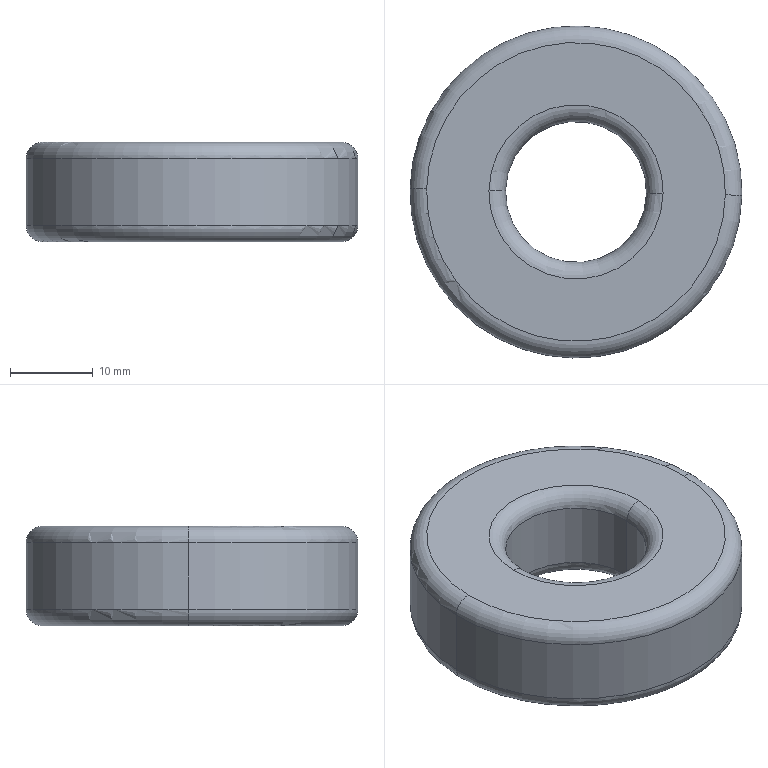Component | SolidWorks | NewCurveBender6203Bearing-DoubleWheel-1 | 1 solid | 14 faces | box 40 x 40 x 12 mm | volume 12048 mm3 | torus 8 | cylinder 4 | plane 2 | commonest cylinder face diameters 17 x2 40 x2
build123d program:
from build123d import *

# Parameters (mm, degrees)
SKETCH1_R           = 20
SKETCH1_R_2         = 8.5
BOSS_EXTRUDE1_DEPTH = 12
FILLET1_R           = 2


with BuildPart() as part:
    # Sketch1 → Boss-Extrude1 (new body)
    with BuildSketch(Plane.XY):
        Circle(SKETCH1_R)
        Circle(SKETCH1_R_2, mode=Mode.SUBTRACT)
    extrude(amount=BOSS_EXTRUDE1_DEPTH)

    # Fillet1
    fillet1_edges = [part.edges().sort_by_distance(p)[0] for p in [
        (-20, 0, 0),
        (-20, 0, 12),
        (-8.5, 0, 0),
        (-8.5, 0, 12),
    ]]
    fillet(fillet1_edges, radius=FILLET1_R)


solid = part.part

# Placed as in the assembly
solid = solid.moved(Location((0, -50.5, 47), (0, 0, 0)))
STEP:
#1=COLOUR_RGB('',0.7922,0.8196,0.9333);
#2=FILL_AREA_STYLE_COLOUR('',#1);
#3=FILL_AREA_STYLE('',(#2));
#4=SURFACE_STYLE_FILL_AREA(#3);
#5=SURFACE_SIDE_STYLE('',(#4));
#6=SURFACE_STYLE_USAGE(.BOTH.,#5);
#7=PRESENTATION_STYLE_ASSIGNMENT((#6));
#8=CARTESIAN_POINT('',(-0.7872,-1.973,2.244));
#9=VERTEX_POINT('',#8);
#10=CARTESIAN_POINT('',(0.7872,-2.004,2.244));
#11=VERTEX_POINT('',#10);
#12=CARTESIAN_POINT('',(0.,-1.988,2.244));
#13=DIRECTION('',(0.,0.,-1.));
#14=DIRECTION('',(0.9998,-0.01988,0.));
#15=AXIS2_PLACEMENT_3D('',#12,#13,#14);
#16=CIRCLE('',#15,0.7874);
#17=EDGE_CURVE('',#9,#11,#16,.T.);
#18=ORIENTED_EDGE('',*,*,#17,.F.);
#19=CARTESIAN_POINT('',(-0.7085,-1.974,2.323));
#20=VERTEX_POINT('',#19);
#21=CARTESIAN_POINT('',(-0.7085,-1.974,2.244));
#22=DIRECTION('',(0.01988,0.9998,0.));
#23=DIRECTION('',(-0.9998,0.01988,0.));
#24=AXIS2_PLACEMENT_3D('',#21,#22,#23);
#25=CIRCLE('',#24,0.07874);
#26=EDGE_CURVE('',#9,#20,#25,.T.);
#27=ORIENTED_EDGE('',*,*,#26,.T.);
#28=CARTESIAN_POINT('',(0.7085,-2.002,2.323));
#29=VERTEX_POINT('',#28);
#30=CARTESIAN_POINT('',(0.,-1.988,2.323));
#31=DIRECTION('',(0.,0.,1.));
#32=DIRECTION('',(0.9998,-0.01988,0.));
#33=AXIS2_PLACEMENT_3D('',#30,#31,#32);
#34=CIRCLE('',#33,0.7087);
#35=EDGE_CURVE('',#29,#20,#34,.T.);
#36=ORIENTED_EDGE('',*,*,#35,.F.);
#37=CARTESIAN_POINT('',(0.7085,-2.002,2.244));
#38=DIRECTION('',(-0.01988,-0.9998,0.));
#39=DIRECTION('',(0.9998,-0.01988,0.));
#40=AXIS2_PLACEMENT_3D('',#37,#38,#39);
#41=CIRCLE('',#40,0.07874);
#42=EDGE_CURVE('',#11,#29,#41,.T.);
#43=ORIENTED_EDGE('',*,*,#42,.F.);
#44=EDGE_LOOP('',(#18,#27,#36,#43));
#45=FACE_OUTER_BOUND('',#44,.T.);
#46=CARTESIAN_POINT('',(0.,-1.988,2.244));
#47=DIRECTION('',(0.,0.,1.));
#48=DIRECTION('',(0.9998,-0.01988,0.));
#49=AXIS2_PLACEMENT_3D('',#46,#47,#48);
#50=TOROIDAL_SURFACE('',#49,0.7087,0.07874);
#51=ADVANCED_FACE('',(#45),#50,.T.);
#52=CARTESIAN_POINT('',(-0.4133,-1.98,2.323));
#53=VERTEX_POINT('',#52);
#54=CARTESIAN_POINT('',(0.4133,-1.996,2.323));
#55=VERTEX_POINT('',#54);
#56=CARTESIAN_POINT('',(0.,-1.988,2.323));
#57=DIRECTION('',(0.,0.,-1.));
#58=DIRECTION('',(0.9998,-0.01988,0.));
#59=AXIS2_PLACEMENT_3D('',#56,#57,#58);
#60=CIRCLE('',#59,0.4134);
#61=EDGE_CURVE('',#53,#55,#60,.T.);
#62=ORIENTED_EDGE('',*,*,#61,.F.);
#63=CARTESIAN_POINT('',(-0.3346,-1.982,2.244));
#64=VERTEX_POINT('',#63);
#65=CARTESIAN_POINT('',(-0.4133,-1.98,2.244));
#66=DIRECTION('',(0.01988,0.9998,0.));
#67=DIRECTION('',(-0.9998,0.01988,0.));
#68=AXIS2_PLACEMENT_3D('',#65,#66,#67);
#69=CIRCLE('',#68,0.07874);
#70=EDGE_CURVE('',#53,#64,#69,.T.);
#71=ORIENTED_EDGE('',*,*,#70,.T.);
#72=CARTESIAN_POINT('',(0.3346,-1.995,2.244));
#73=VERTEX_POINT('',#72);
#74=CARTESIAN_POINT('',(0.,-1.988,2.244));
#75=DIRECTION('',(0.,0.,1.));
#76=DIRECTION('',(0.9998,-0.01988,0.));
#77=AXIS2_PLACEMENT_3D('',#74,#75,#76);
#78=CIRCLE('',#77,0.3346);
#79=EDGE_CURVE('',#73,#64,#78,.T.);
#80=ORIENTED_EDGE('',*,*,#79,.F.);
#81=CARTESIAN_POINT('',(0.4133,-1.996,2.244));
#82=DIRECTION('',(-0.01988,-0.9998,0.));
#83=DIRECTION('',(0.9998,-0.01988,0.));
#84=AXIS2_PLACEMENT_3D('',#81,#82,#83);
#85=CIRCLE('',#84,0.07874);
#86=EDGE_CURVE('',#55,#73,#85,.T.);
#87=ORIENTED_EDGE('',*,*,#86,.F.);
#88=EDGE_LOOP('',(#62,#71,#80,#87));
#89=FACE_OUTER_BOUND('',#88,.T.);
#90=CARTESIAN_POINT('',(0.,-1.988,2.244));
#91=DIRECTION('',(0.,0.,1.));
#92=DIRECTION('',(0.9998,-0.01988,0.));
#93=AXIS2_PLACEMENT_3D('',#90,#91,#92);
#94=TOROIDAL_SURFACE('',#93,0.4134,0.07874);
#95=ADVANCED_FACE('',(#89),#94,.T.);
#96=CARTESIAN_POINT('',(-0.7085,-1.974,1.85));
#97=VERTEX_POINT('',#96);
#98=CARTESIAN_POINT('',(0.7085,-2.002,1.85));
#99=VERTEX_POINT('',#98);
#100=CARTESIAN_POINT('',(0.,-1.988,1.85));
#101=DIRECTION('',(0.,0.,-1.));
#102=DIRECTION('',(0.9998,-0.01988,0.));
#103=AXIS2_PLACEMENT_3D('',#100,#101,#102);
#104=CIRCLE('',#103,0.7087);
#105=EDGE_CURVE('',#97,#99,#104,.T.);
#106=ORIENTED_EDGE('',*,*,#105,.F.);
#107=CARTESIAN_POINT('',(-0.7872,-1.973,1.929));
#108=VERTEX_POINT('',#107);
#109=CARTESIAN_POINT('',(-0.7085,-1.974,1.929));
#110=DIRECTION('',(0.01988,0.9998,0.));
#111=DIRECTION('',(-0.9998,0.01988,0.));
#112=AXIS2_PLACEMENT_3D('',#109,#110,#111);
#113=CIRCLE('',#112,0.07874);
#114=EDGE_CURVE('',#97,#108,#113,.T.);
#115=ORIENTED_EDGE('',*,*,#114,.T.);
#116=CARTESIAN_POINT('',(0.7872,-2.004,1.929));
#117=VERTEX_POINT('',#116);
#118=CARTESIAN_POINT('',(0.,-1.988,1.929));
#119=DIRECTION('',(0.,0.,1.));
#120=DIRECTION('',(0.9998,-0.01988,0.));
#121=AXIS2_PLACEMENT_3D('',#118,#119,#120);
#122=CIRCLE('',#121,0.7874);
#123=EDGE_CURVE('',#117,#108,#122,.T.);
#124=ORIENTED_EDGE('',*,*,#123,.F.);
#125=CARTESIAN_POINT('',(0.7085,-2.002,1.929));
#126=DIRECTION('',(-0.01988,-0.9998,0.));
#127=DIRECTION('',(0.9998,-0.01988,0.));
#128=AXIS2_PLACEMENT_3D('',#125,#126,#127);
#129=CIRCLE('',#128,0.07874);
#130=EDGE_CURVE('',#99,#117,#129,.T.);
#131=ORIENTED_EDGE('',*,*,#130,.F.);
#132=EDGE_LOOP('',(#106,#115,#124,#131));
#133=FACE_OUTER_BOUND('',#132,.T.);
#134=CARTESIAN_POINT('',(0.,-1.988,1.929));
#135=DIRECTION('',(0.,0.,1.));
#136=DIRECTION('',(0.9998,-0.01988,0.));
#137=AXIS2_PLACEMENT_3D('',#134,#135,#136);
#138=TOROIDAL_SURFACE('',#137,0.7087,0.07874);
#139=ADVANCED_FACE('',(#133),#138,.T.);
#140=CARTESIAN_POINT('',(-0.3346,-1.982,1.929));
#141=VERTEX_POINT('',#140);
#142=CARTESIAN_POINT('',(0.3346,-1.995,1.929));
#143=VERTEX_POINT('',#142);
#144=CARTESIAN_POINT('',(0.,-1.988,1.929));
#145=DIRECTION('',(0.,0.,-1.));
#146=DIRECTION('',(0.9998,-0.01988,0.));
#147=AXIS2_PLACEMENT_3D('',#144,#145,#146);
#148=CIRCLE('',#147,0.3346);
#149=EDGE_CURVE('',#141,#143,#148,.T.);
#150=ORIENTED_EDGE('',*,*,#149,.F.);
#151=CARTESIAN_POINT('',(-0.4133,-1.98,1.85));
#152=VERTEX_POINT('',#151);
#153=CARTESIAN_POINT('',(-0.4133,-1.98,1.929));
#154=DIRECTION('',(0.01988,0.9998,0.));
#155=DIRECTION('',(-0.9998,0.01988,0.));
#156=AXIS2_PLACEMENT_3D('',#153,#154,#155);
#157=CIRCLE('',#156,0.07874);
#158=EDGE_CURVE('',#141,#152,#157,.T.);
#159=ORIENTED_EDGE('',*,*,#158,.T.);
#160=CARTESIAN_POINT('',(0.4133,-1.996,1.85));
#161=VERTEX_POINT('',#160);
#162=CARTESIAN_POINT('',(0.,-1.988,1.85));
#163=DIRECTION('',(0.,0.,1.));
#164=DIRECTION('',(0.9998,-0.01988,0.));
#165=AXIS2_PLACEMENT_3D('',#162,#163,#164);
#166=CIRCLE('',#165,0.4134);
#167=EDGE_CURVE('',#161,#152,#166,.T.);
#168=ORIENTED_EDGE('',*,*,#167,.F.);
#169=CARTESIAN_POINT('',(0.4133,-1.996,1.929));
#170=DIRECTION('',(-0.01988,-0.9998,0.));
#171=DIRECTION('',(0.9998,-0.01988,0.));
#172=AXIS2_PLACEMENT_3D('',#169,#170,#171);
#173=CIRCLE('',#172,0.07874);
#174=EDGE_CURVE('',#143,#161,#173,.T.);
#175=ORIENTED_EDGE('',*,*,#174,.F.);
#176=EDGE_LOOP('',(#150,#159,#168,#175));
#177=FACE_OUTER_BOUND('',#176,.T.);
#178=CARTESIAN_POINT('',(0.,-1.988,1.929));
#179=DIRECTION('',(0.,0.,1.));
#180=DIRECTION('',(0.9998,-0.01988,0.));
#181=AXIS2_PLACEMENT_3D('',#178,#179,#180);
#182=TOROIDAL_SURFACE('',#181,0.4134,0.07874);
#183=ADVANCED_FACE('',(#177),#182,.T.);
#184=CARTESIAN_POINT('',(0.,-1.988,2.244));
#185=DIRECTION('',(0.,0.,1.));
#186=DIRECTION('',(0.9998,-0.01988,0.));
#187=AXIS2_PLACEMENT_3D('',#184,#185,#186);
#188=CIRCLE('',#187,0.3346);
#189=EDGE_CURVE('',#64,#73,#188,.T.);
#190=ORIENTED_EDGE('',*,*,#189,.T.);
#191=CARTESIAN_POINT('',(0.3346,-1.995,2.323));
#192=DIRECTION('',(0.,0.,-1.));
#193=VECTOR('',#192,39.37);
#194=LINE('',#191,#193);
#195=EDGE_CURVE('',#73,#143,#194,.T.);
#196=ORIENTED_EDGE('',*,*,#195,.T.);
#197=CARTESIAN_POINT('',(0.,-1.988,1.929));
#198=DIRECTION('',(0.,0.,-1.));
#199=DIRECTION('',(0.9998,-0.01988,0.));
#200=AXIS2_PLACEMENT_3D('',#197,#198,#199);
#201=CIRCLE('',#200,0.3346);
#202=EDGE_CURVE('',#143,#141,#201,.T.);
#203=ORIENTED_EDGE('',*,*,#202,.T.);
#204=CARTESIAN_POINT('',(-0.3346,-1.982,2.323));
#205=DIRECTION('',(0.,0.,-1.));
#206=VECTOR('',#205,39.37);
#207=LINE('',#204,#206);
#208=EDGE_CURVE('',#64,#141,#207,.T.);
#209=ORIENTED_EDGE('',*,*,#208,.F.);
#210=EDGE_LOOP('',(#190,#196,#203,#209));
#211=FACE_OUTER_BOUND('',#210,.T.);
#212=CARTESIAN_POINT('',(0.,-1.988,2.323));
#213=DIRECTION('',(0.,0.,-1.));
#214=DIRECTION('',(-0.9998,0.01988,0.));
#215=AXIS2_PLACEMENT_3D('',#212,#213,#214);
#216=CYLINDRICAL_SURFACE('',#215,0.3346);
#217=ADVANCED_FACE('',(#211),#216,.F.);
#218=ORIENTED_EDGE('',*,*,#17,.T.);
#219=CARTESIAN_POINT('',(0.7872,-2.004,2.323));
#220=DIRECTION('',(0.,0.,-1.));
#221=VECTOR('',#220,39.37);
#222=LINE('',#219,#221);
#223=EDGE_CURVE('',#11,#117,#222,.T.);
#224=ORIENTED_EDGE('',*,*,#223,.T.);
#225=ORIENTED_EDGE('',*,*,#123,.T.);
#226=CARTESIAN_POINT('',(-0.7872,-1.973,2.323));
#227=DIRECTION('',(0.,0.,-1.));
#228=VECTOR('',#227,39.37);
#229=LINE('',#226,#228);
#230=EDGE_CURVE('',#9,#108,#229,.T.);
#231=ORIENTED_EDGE('',*,*,#230,.F.);
#232=EDGE_LOOP('',(#218,#224,#225,#231));
#233=FACE_OUTER_BOUND('',#232,.T.);
#234=CARTESIAN_POINT('',(0.,-1.988,2.323));
#235=DIRECTION('',(0.,0.,-1.));
#236=DIRECTION('',(-0.9998,0.01988,0.));
#237=AXIS2_PLACEMENT_3D('',#234,#235,#236);
#238=CYLINDRICAL_SURFACE('',#237,0.7874);
#239=ADVANCED_FACE('',(#233),#238,.T.);
#240=CARTESIAN_POINT('',(0.,-1.988,2.323));
#241=DIRECTION('',(0.,0.,-1.));
#242=DIRECTION('',(0.9998,-0.01988,0.));
#243=AXIS2_PLACEMENT_3D('',#240,#241,#242);
#244=CIRCLE('',#243,0.4134);
#245=EDGE_CURVE('',#55,#53,#244,.T.);
#246=ORIENTED_EDGE('',*,*,#245,.T.);
#247=ORIENTED_EDGE('',*,*,#61,.T.);
#248=EDGE_LOOP('',(#246,#247));
#249=FACE_BOUND('',#248,.T.);
#250=ORIENTED_EDGE('',*,*,#35,.T.);
#251=CARTESIAN_POINT('',(0.,-1.988,2.323));
#252=DIRECTION('',(0.,0.,1.));
#253=DIRECTION('',(0.9998,-0.01988,0.));
#254=AXIS2_PLACEMENT_3D('',#251,#252,#253);
#255=CIRCLE('',#254,0.7087);
#256=EDGE_CURVE('',#20,#29,#255,.T.);
#257=ORIENTED_EDGE('',*,*,#256,.T.);
#258=EDGE_LOOP('',(#250,#257));
#259=FACE_OUTER_BOUND('',#258,.T.);
#260=CARTESIAN_POINT('',(0.,-1.988,2.323));
#261=DIRECTION('',(0.,0.,1.));
#262=DIRECTION('',(0.9998,-0.01988,0.));
#263=AXIS2_PLACEMENT_3D('',#260,#261,#262);
#264=PLANE('',#263);
#265=ADVANCED_FACE('',(#249,#259),#264,.T.);
#266=ORIENTED_EDGE('',*,*,#167,.T.);
#267=CARTESIAN_POINT('',(0.,-1.988,1.85));
#268=DIRECTION('',(0.,0.,1.));
#269=DIRECTION('',(0.9998,-0.01988,0.));
#270=AXIS2_PLACEMENT_3D('',#267,#268,#269);
#271=CIRCLE('',#270,0.4134);
#272=EDGE_CURVE('',#152,#161,#271,.T.);
#273=ORIENTED_EDGE('',*,*,#272,.T.);
#274=EDGE_LOOP('',(#266,#273));
#275=FACE_BOUND('',#274,.T.);
#276=CARTESIAN_POINT('',(0.,-1.988,1.85));
#277=DIRECTION('',(0.,0.,-1.));
#278=DIRECTION('',(0.9998,-0.01988,0.));
#279=AXIS2_PLACEMENT_3D('',#276,#277,#278);
#280=CIRCLE('',#279,0.7087);
#281=EDGE_CURVE('',#99,#97,#280,.T.);
#282=ORIENTED_EDGE('',*,*,#281,.T.);
#283=ORIENTED_EDGE('',*,*,#105,.T.);
#284=EDGE_LOOP('',(#282,#283));
#285=FACE_OUTER_BOUND('',#284,.T.);
#286=CARTESIAN_POINT('',(0.,-1.988,1.85));
#287=DIRECTION('',(0.,0.,1.));
#288=DIRECTION('',(0.9998,-0.01988,0.));
#289=AXIS2_PLACEMENT_3D('',#286,#287,#288);
#290=PLANE('',#289);
#291=ADVANCED_FACE('',(#275,#285),#290,.F.);
#292=ORIENTED_EDGE('',*,*,#223,.F.);
#293=CARTESIAN_POINT('',(0.,-1.988,2.244));
#294=DIRECTION('',(0.,0.,-1.));
#295=DIRECTION('',(0.9998,-0.01988,0.));
#296=AXIS2_PLACEMENT_3D('',#293,#294,#295);
#297=CIRCLE('',#296,0.7874);
#298=EDGE_CURVE('',#11,#9,#297,.T.);
#299=ORIENTED_EDGE('',*,*,#298,.T.);
#300=ORIENTED_EDGE('',*,*,#230,.T.);
#301=CARTESIAN_POINT('',(0.,-1.988,1.929));
#302=DIRECTION('',(0.,0.,1.));
#303=DIRECTION('',(0.9998,-0.01988,0.));
#304=AXIS2_PLACEMENT_3D('',#301,#302,#303);
#305=CIRCLE('',#304,0.7874);
#306=EDGE_CURVE('',#108,#117,#305,.T.);
#307=ORIENTED_EDGE('',*,*,#306,.T.);
#308=EDGE_LOOP('',(#292,#299,#300,#307));
#309=FACE_OUTER_BOUND('',#308,.T.);
#310=CARTESIAN_POINT('',(0.,-1.988,2.323));
#311=DIRECTION('',(0.,0.,-1.));
#312=DIRECTION('',(-0.9998,0.01988,0.));
#313=AXIS2_PLACEMENT_3D('',#310,#311,#312);
#314=CYLINDRICAL_SURFACE('',#313,0.7874);
#315=ADVANCED_FACE('',(#309),#314,.T.);
#316=ORIENTED_EDGE('',*,*,#195,.F.);
#317=ORIENTED_EDGE('',*,*,#79,.T.);
#318=ORIENTED_EDGE('',*,*,#208,.T.);
#319=ORIENTED_EDGE('',*,*,#149,.T.);
#320=EDGE_LOOP('',(#316,#317,#318,#319));
#321=FACE_OUTER_BOUND('',#320,.T.);
#322=CARTESIAN_POINT('',(0.,-1.988,2.323));
#323=DIRECTION('',(0.,0.,-1.));
#324=DIRECTION('',(-0.9998,0.01988,0.));
#325=AXIS2_PLACEMENT_3D('',#322,#323,#324);
#326=CYLINDRICAL_SURFACE('',#325,0.3346);
#327=ADVANCED_FACE('',(#321),#326,.F.);
#328=ORIENTED_EDGE('',*,*,#158,.F.);
#329=ORIENTED_EDGE('',*,*,#202,.F.);
#330=ORIENTED_EDGE('',*,*,#174,.T.);
#331=ORIENTED_EDGE('',*,*,#272,.F.);
#332=EDGE_LOOP('',(#328,#329,#330,#331));
#333=FACE_OUTER_BOUND('',#332,.T.);
#334=CARTESIAN_POINT('',(0.,-1.988,1.929));
#335=DIRECTION('',(0.,0.,1.));
#336=DIRECTION('',(0.9998,-0.01988,0.));
#337=AXIS2_PLACEMENT_3D('',#334,#335,#336);
#338=TOROIDAL_SURFACE('',#337,0.4134,0.07874);
#339=ADVANCED_FACE('',(#333),#338,.T.);
#340=ORIENTED_EDGE('',*,*,#114,.F.);
#341=ORIENTED_EDGE('',*,*,#281,.F.);
#342=ORIENTED_EDGE('',*,*,#130,.T.);
#343=ORIENTED_EDGE('',*,*,#306,.F.);
#344=EDGE_LOOP('',(#340,#341,#342,#343));
#345=FACE_OUTER_BOUND('',#344,.T.);
#346=CARTESIAN_POINT('',(0.,-1.988,1.929));
#347=DIRECTION('',(0.,0.,1.));
#348=DIRECTION('',(0.9998,-0.01988,0.));
#349=AXIS2_PLACEMENT_3D('',#346,#347,#348);
#350=TOROIDAL_SURFACE('',#349,0.7087,0.07874);
#351=ADVANCED_FACE('',(#345),#350,.T.);
#352=ORIENTED_EDGE('',*,*,#70,.F.);
#353=ORIENTED_EDGE('',*,*,#245,.F.);
#354=ORIENTED_EDGE('',*,*,#86,.T.);
#355=ORIENTED_EDGE('',*,*,#189,.F.);
#356=EDGE_LOOP('',(#352,#353,#354,#355));
#357=FACE_OUTER_BOUND('',#356,.T.);
#358=CARTESIAN_POINT('',(0.,-1.988,2.244));
#359=DIRECTION('',(0.,0.,1.));
#360=DIRECTION('',(0.9998,-0.01988,0.));
#361=AXIS2_PLACEMENT_3D('',#358,#359,#360);
#362=TOROIDAL_SURFACE('',#361,0.4134,0.07874);
#363=ADVANCED_FACE('',(#357),#362,.T.);
#364=ORIENTED_EDGE('',*,*,#26,.F.);
#365=ORIENTED_EDGE('',*,*,#298,.F.);
#366=ORIENTED_EDGE('',*,*,#42,.T.);
#367=ORIENTED_EDGE('',*,*,#256,.F.);
#368=EDGE_LOOP('',(#364,#365,#366,#367));
#369=FACE_OUTER_BOUND('',#368,.T.);
#370=CARTESIAN_POINT('',(0.,-1.988,2.244));
#371=DIRECTION('',(0.,0.,1.));
#372=DIRECTION('',(0.9998,-0.01988,0.));
#373=AXIS2_PLACEMENT_3D('',#370,#371,#372);
#374=TOROIDAL_SURFACE('',#373,0.7087,0.07874);
#375=ADVANCED_FACE('',(#369),#374,.T.);
#376=CLOSED_SHELL('',(#51,#95,#139,#183,#217,#239,#265,#291,#315,#327,#339,#351,#363,#375));
#377=MANIFOLD_SOLID_BREP('',#376);
#378=STYLED_ITEM('',(#7),#377);
#379=PRESENTATION_LAYER_ASSIGNMENT('','',(#378));
#380=CARTESIAN_POINT('',(0.,0.,0.));
#381=DIRECTION('',(0.,0.,1.));
#382=DIRECTION('',(1.,0.,0.));
#383=AXIS2_PLACEMENT_3D('',#380,#381,#382);
#384=(LENGTH_UNIT()NAMED_UNIT(*)SI_UNIT($,.METRE.));
#385=LENGTH_MEASURE_WITH_UNIT(LENGTH_MEASURE(0.0254),#384);
#386=DIMENSIONAL_EXPONENTS(1.,0.,0.,0.,0.,0.,0.);
#387=(CONVERSION_BASED_UNIT('',#385)LENGTH_UNIT()NAMED_UNIT(#386));
#388=UNCERTAINTY_MEASURE_WITH_UNIT(LENGTH_MEASURE(0.00001),#387,'','');
#389=(NAMED_UNIT(*)PLANE_ANGLE_UNIT()SI_UNIT($,.RADIAN.));
#390=(NAMED_UNIT(*)SI_UNIT($,.STERADIAN.)SOLID_ANGLE_UNIT());
#391=(GEOMETRIC_REPRESENTATION_CONTEXT(3)GLOBAL_UNCERTAINTY_ASSIGNED_CONTEXT((#388))GLOBAL_UNIT_ASSIGNED_CONTEXT((#387,#389,#390))REPRESENTATION_CONTEXT('',''));
#392=ADVANCED_BREP_SHAPE_REPRESENTATION('',(#377,#383),#391);
#393=(LENGTH_UNIT()NAMED_UNIT(*)SI_UNIT($,.METRE.));
#394=LENGTH_MEASURE_WITH_UNIT(LENGTH_MEASURE(0.0254),#393);
#395=DIMENSIONAL_EXPONENTS(1.,0.,0.,0.,0.,0.,0.);
#396=(CONVERSION_BASED_UNIT('',#394)LENGTH_UNIT()NAMED_UNIT(#395));
#397=UNCERTAINTY_MEASURE_WITH_UNIT(LENGTH_MEASURE(0.00001),#396,'','');
#398=(NAMED_UNIT(*)PLANE_ANGLE_UNIT()SI_UNIT($,.RADIAN.));
#399=(NAMED_UNIT(*)SI_UNIT($,.STERADIAN.)SOLID_ANGLE_UNIT());
#400=(GEOMETRIC_REPRESENTATION_CONTEXT(3)GLOBAL_UNCERTAINTY_ASSIGNED_CONTEXT((#397))GLOBAL_UNIT_ASSIGNED_CONTEXT((#396,#398,#399))REPRESENTATION_CONTEXT('',''));
#401=MECHANICAL_DESIGN_GEOMETRIC_PRESENTATION_REPRESENTATION('',(#378),#400);